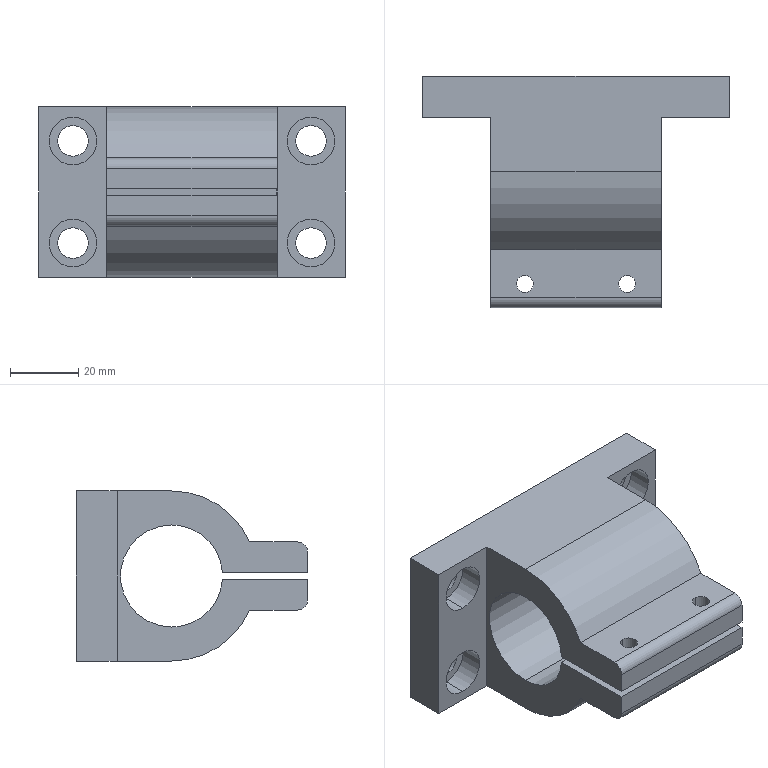Component | SolidWorks | 36LeadScrewNut-1 | 1 solid | 57 faces | volume 114100 mm3 | cylinder 31 | plane 19 | cone 7 | commonest cylinder face diameters 14 x8 9 x8 5 x4 7 x4 30 x3 50 x2 6 x2